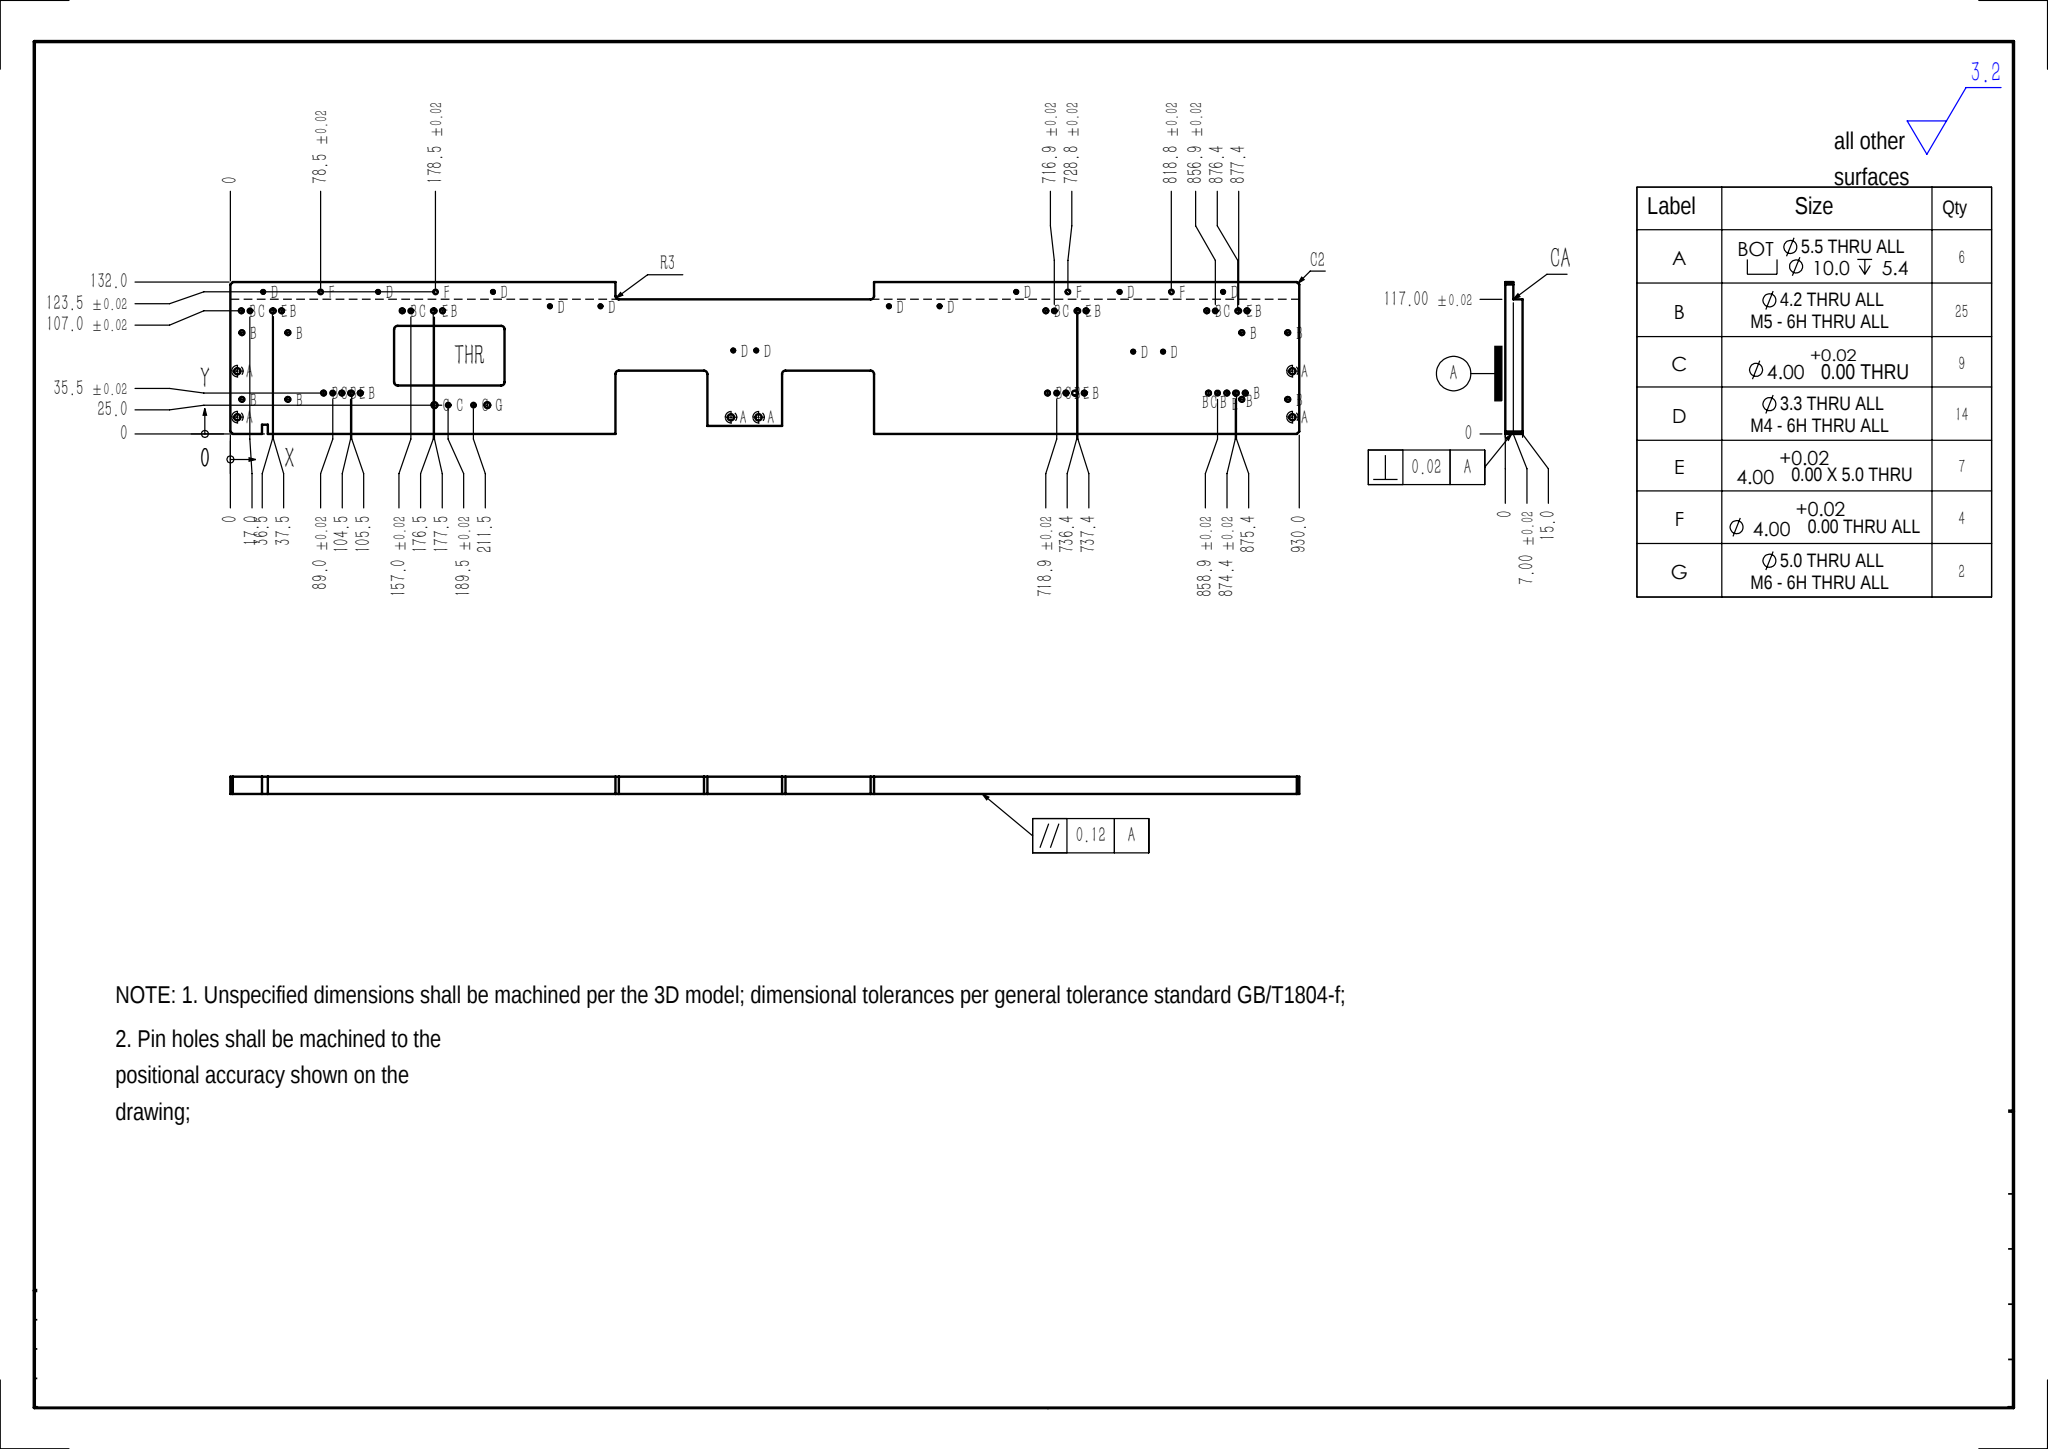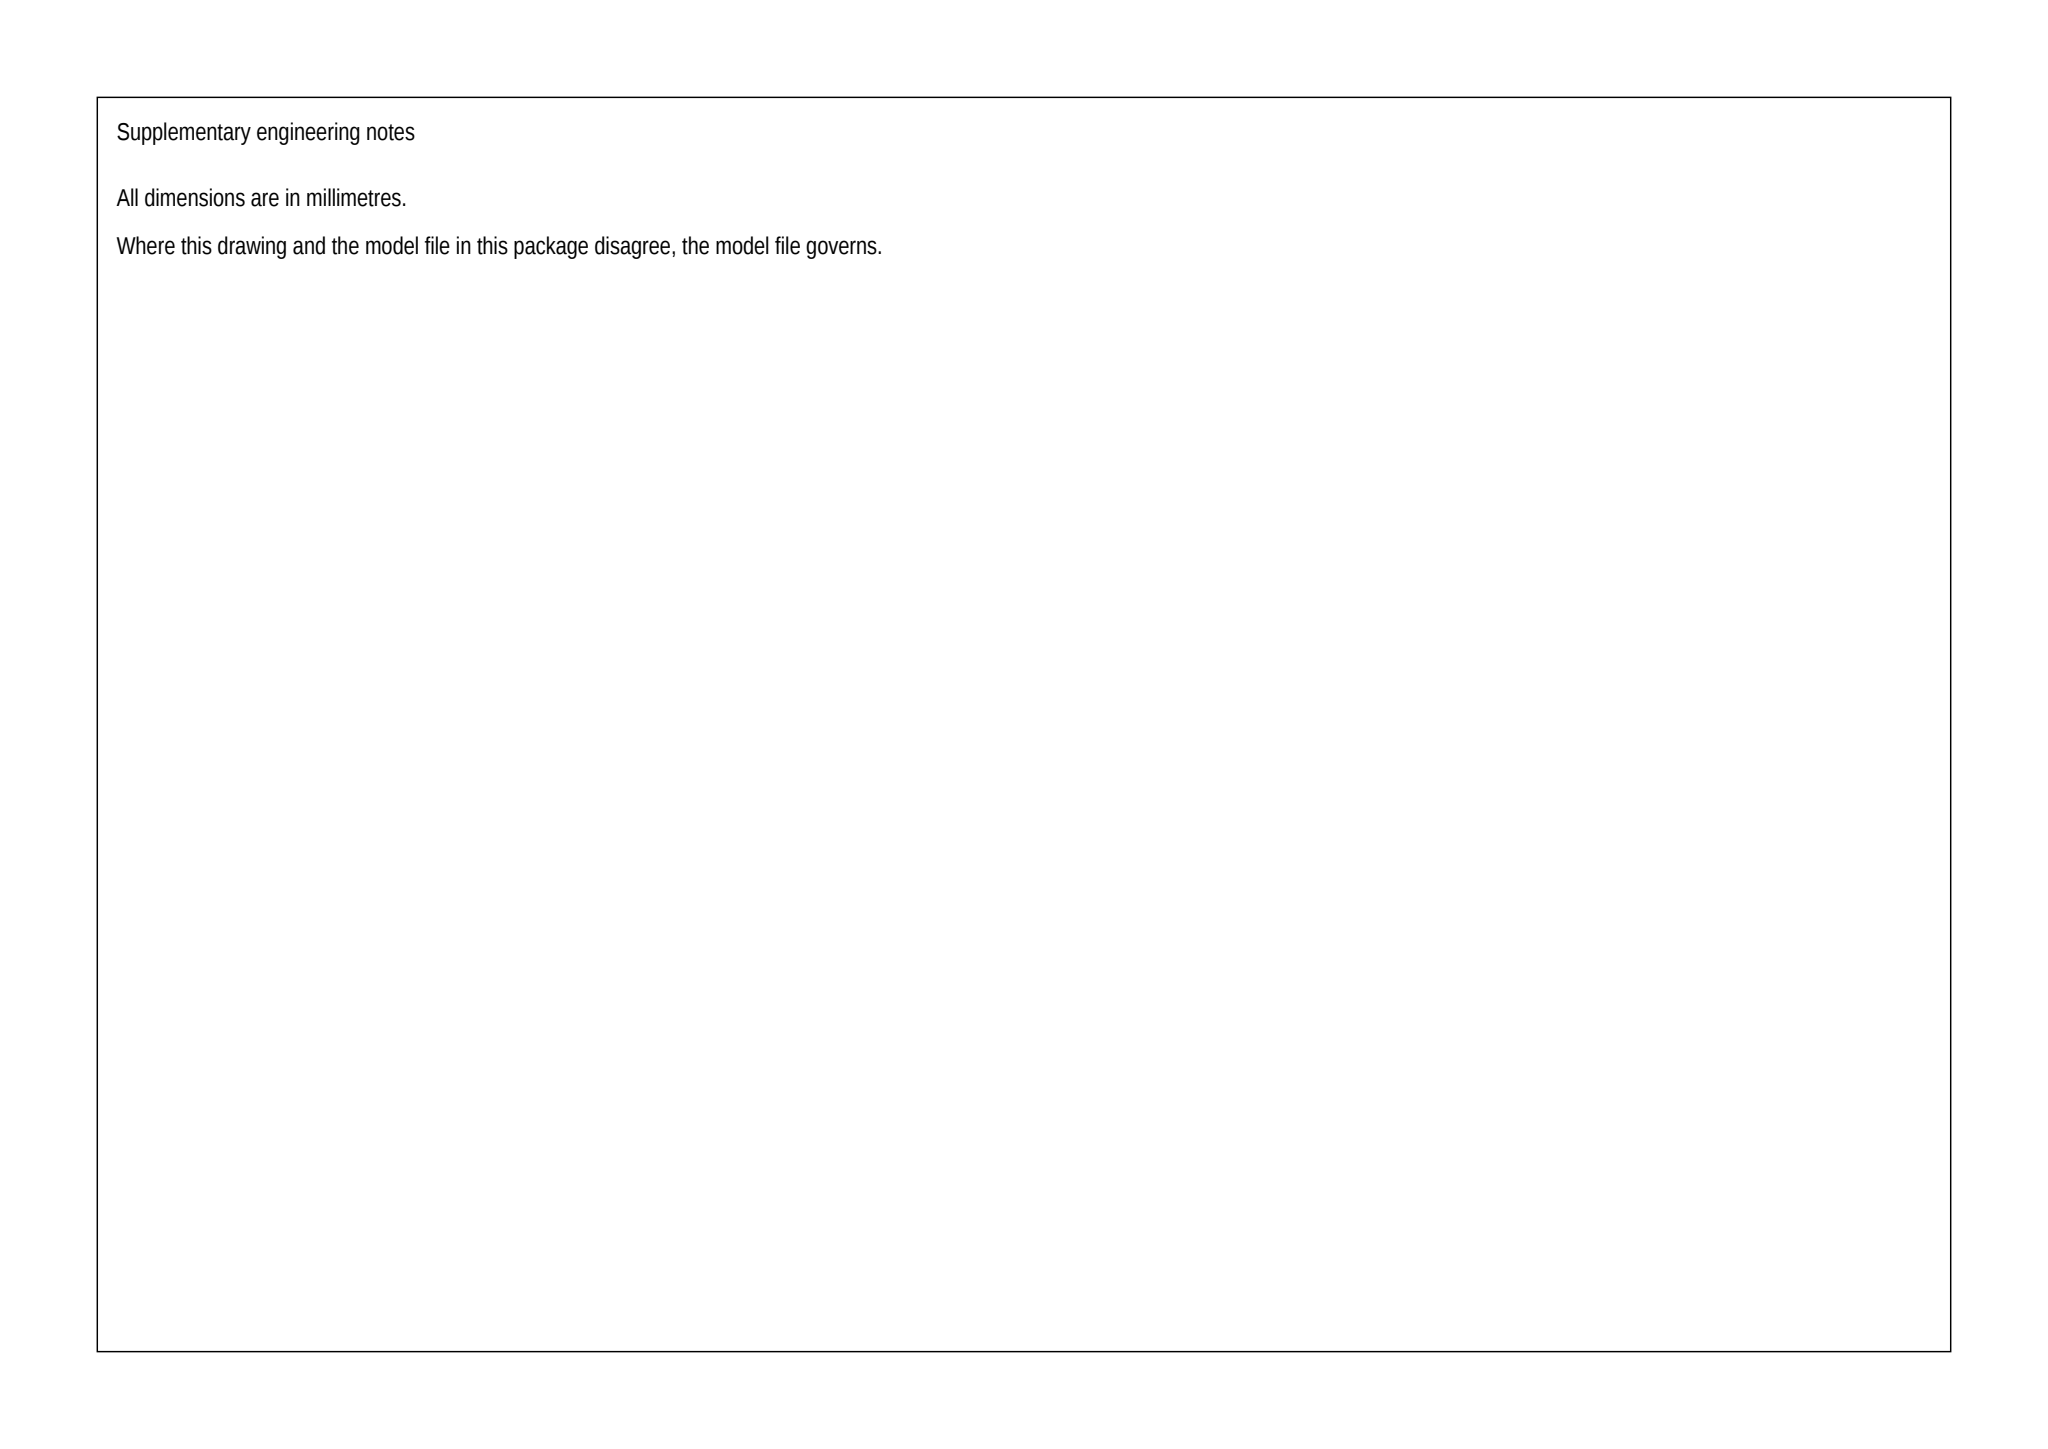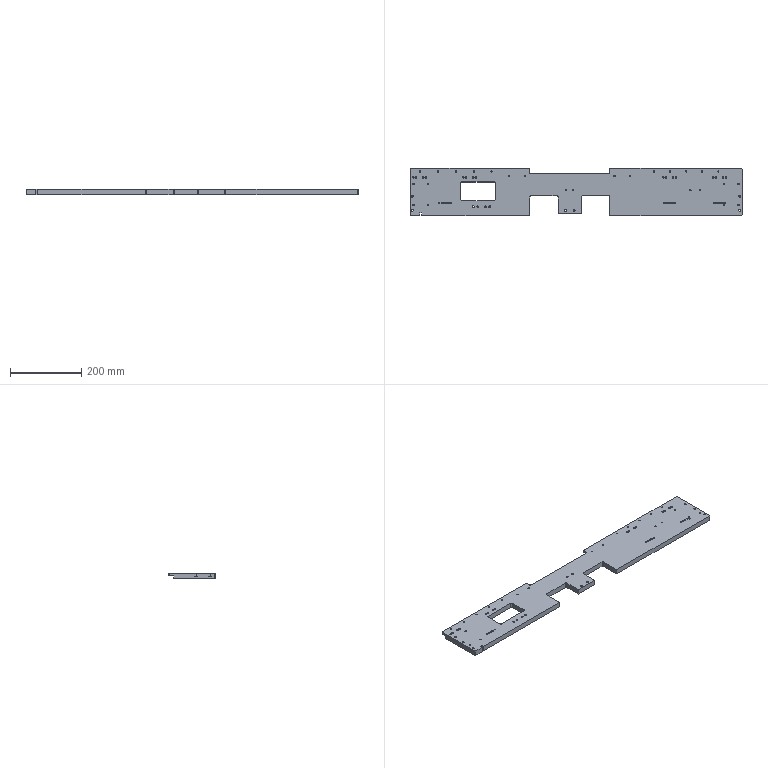Part | SolidWorks | mm | 1 solid | 215 faces | box 930 x 132 x 15 mm | volume 1477170 mm3 | cylinder 163 | plane 52 | commonest cylinder face diameters 4.2 x50 4 x47 3.3 x28 10 x12 5.5 x12 6 x10 5 x4
build123d program:
from build123d import *

# Parameters (mm, degrees)
SKETCH1_W                                       = 930
SKETCH1_H                                       = 132
BOSS_EXTRUDE1_DEPTH                             = 15
SKETCH3_W                                       = 930
SKETCH3_H                                       = 8
CUT_EXTRUDE2_DEPTH                              = 15
SKETCH19_W                                      = 80
SKETCH19_H                                      = 55
SKETCH19_W_2                                    = 225
SKETCH19_H_2                                    = 15
CUT_EXTRUDE3_DEPTH                              = 470.9
SKETCH20_W                                      = 65
SKETCH20_H                                      = 7
CUT_EXTRUDE4_DEPTH                              = 470.9
SKETCH22_W                                      = 96
SKETCH22_H                                      = 52
CUT_EXTRUDE5_DEPTH                              = 470.9
FILLET1_R                                       = 3
M4_TAPPED_HOLE1_D                               = 3.3
M5_TAPPED_HOLE1_D                               = 4.2
M6_TAPPED_HOLE1_D                               = 5
SKETCH29_R                                      = 2
CUT_EXTRUDE6_DEPTH                              = 470.9
CHAMFER1_SIZE                                   = 2
M5_TAPPED_HOLE2_D                               = 4.2
M5_HEX_SOCKET_HEAD_CAP_SCREW_CBORE1_D           = 5.5
M5_HEX_SOCKET_HEAD_CAP_SCREW_CBORE1_CBORE_D     = 10
M5_HEX_SOCKET_HEAD_CAP_SCREW_CBORE1_CBORE_DEPTH = 5.4
M5_HEX_SOCKET_HEAD_CAP_SCREW_CBORE2_D           = 5.5
M5_HEX_SOCKET_HEAD_CAP_SCREW_CBORE2_CBORE_D     = 10
M5_HEX_SOCKET_HEAD_CAP_SCREW_CBORE2_CBORE_DEPTH = 5.4
M5_TAPPED_HOLE3_D                               = 4.2
SKETCH41_W                                      = 5
SKETCH41_H                                      = 8
CUT_EXTRUDE7_DEPTH                              = 470.9
M4_TAPPED_HOLE3_D                               = 3.3
SIZE_MM_DOWEL_HOLE1_D                           = 4


with BuildPart() as part:
    # Sketch1 → Boss-Extrude1 (new body)
    with BuildSketch(Plane.XY):
        Rectangle(SKETCH1_W, SKETCH1_H)
    extrude(amount=BOSS_EXTRUDE1_DEPTH)

    # Sketch3 → Cut-Extrude2 (cut)
    with BuildSketch(Plane(origin=(0, 66, 0), x_dir=(1, 0, 0), z_dir=(0, 1, 0))):
        with Locations((0, -4)):
            Rectangle(SKETCH3_W, SKETCH3_H)
    extrude(amount=-CUT_EXTRUDE2_DEPTH, mode=Mode.SUBTRACT)

    # Sketch19 → Cut-Extrude3 (cut, through all)
    with BuildSketch(Plane.XY.offset(15)):
        with Locations((-90, -38.5)):
            Rectangle(SKETCH19_W, SKETCH19_H)
        with Locations((55, -38.5)):
            Rectangle(SKETCH19_W, SKETCH19_H)
        with Locations((-17.5, 58.5)):
            Rectangle(SKETCH19_W_2, SKETCH19_H_2)
    extrude(amount=-CUT_EXTRUDE3_DEPTH, mode=Mode.SUBTRACT)

    # Sketch20 → Cut-Extrude4 (cut, through all)
    with BuildSketch(Plane.XY.offset(15)):
        with Locations((-17.5, -62.5)):
            Rectangle(SKETCH20_W, SKETCH20_H)
    extrude(amount=-CUT_EXTRUDE4_DEPTH, mode=Mode.SUBTRACT)

    # Sketch22 → Cut-Extrude5 (cut, through all)
    with BuildSketch(Plane.XY.offset(15)):
        with Locations((-274.5, 2)):
            Rectangle(SKETCH22_W, SKETCH22_H)
    extrude(amount=-CUT_EXTRUDE5_DEPTH, mode=Mode.SUBTRACT)

    # Fillet1
    fillet1_edges = [part.edges().sort_by_distance(p)[0] for p in [
        (-226.5, 28, 7.5),
        (-226.5, -24, 7.5),
        (95, 51, 11.5),
        (-130, 51, 11.5),
        (15, -11, 7.5),
        (95, -11, 7.5),
        (-130, -11, 7.5),
        (-50, -11, 7.5),
        (-322.5, -24, 7.5),
        (-322.5, 28, 7.5),
    ]]
    fillet(fillet1_edges, radius=FILLET1_R)

    # M4 Tapped Hole1 (through all)
    with Locations(Plane.XY.offset(15)):
        with Locations((-187, 45), (-143, 45), (-27.5, 6.5), (-7.5, 6.5), (108, 45), (152, 45), (320.5, 5.5), (346.5, 5.5)):
            Hole(M4_TAPPED_HOLE1_D / 2)

    # M5 Tapped Hole1 (through all)
    with Locations(Plane.XY.offset(15)):
        with Locations((-384, -30.5), (-368, -30.5), (-352, -30.5), (246, -30.5), (262, -30.5), (278, -30.5), (386, -30.5), (402, -30.5), (418, -30.5)):
            Hole(M5_TAPPED_HOLE1_D / 2)

    # M6 Tapped Hole1 (through all)
    with Locations(Plane.XY.offset(15)):
        with Locations((-287.5, -41), (-241.5, -41)):
            Hole(M6_TAPPED_HOLE1_D / 2)

    # Sketch29 → Cut-Extrude6 (cut, through all)
    with BuildSketch(Plane.XY.offset(15)):
        with Locations((-376, -30.5)):
            Circle(SKETCH29_R)
        with Locations((-275.5, -41)):
            Circle(SKETCH29_R)
        with Locations((-253.5, -41)):
            Circle(SKETCH29_R)
        with Locations((253.922, -30.5)):
            Circle(SKETCH29_R)
        with Locations((393.922, -30.5)):
            Circle(SKETCH29_R)
        with Locations((-448, 41)):
            Circle(SKETCH29_R)
        with Locations((-308, 41)):
            Circle(SKETCH29_R)
        with Locations((251.922, 41)):
            Circle(SKETCH29_R)
        with Locations((391.922, 41)):
            Circle(SKETCH29_R)
        with BuildLine():
            Line((-360.5, -28.5), (-359.5, -28.5))
            ThreePointArc((-359.5, -28.5), (-357.5, -30.5), (-359.5, -32.5))
            Line((-359.5, -32.5), (-360.5, -32.5))
            ThreePointArc((-360.5, -32.5), (-362.5, -30.5), (-360.5, -28.5))
        make_face()
        with BuildLine():
            Line((269.422, -28.5), (270.422, -28.5))
            ThreePointArc((270.422, -28.5), (272.422, -30.5), (270.422, -32.5))
            Line((270.422, -32.5), (269.422, -32.5))
            ThreePointArc((269.422, -32.5), (267.422, -30.5), (269.422, -28.5))
        make_face()
        with BuildLine():
            Line((409.422, -28.5), (410.422, -28.5))
            ThreePointArc((410.422, -28.5), (412.422, -30.5), (410.422, -32.5))
            Line((410.422, -32.5), (409.422, -32.5))
            ThreePointArc((409.422, -32.5), (407.422, -30.5), (409.422, -28.5))
        make_face()
        with BuildLine():
            Line((-428.5, 43), (-427.5, 43))
            ThreePointArc((-427.5, 43), (-425.5, 41), (-427.5, 39))
            Line((-427.5, 39), (-428.5, 39))
            ThreePointArc((-428.5, 39), (-430.5, 41), (-428.5, 43))
        make_face()
        with BuildLine():
            Line((-288.5, 43), (-287.5, 43))
            ThreePointArc((-287.5, 43), (-285.5, 41), (-287.5, 39))
            Line((-287.5, 39), (-288.5, 39))
            ThreePointArc((-288.5, 39), (-290.5, 41), (-288.5, 43))
        make_face()
        with BuildLine():
            Line((271.422, 43), (272.422, 43))
            ThreePointArc((272.422, 43), (274.422, 41), (272.422, 39))
            Line((272.422, 39), (271.422, 39))
            ThreePointArc((271.422, 39), (269.422, 41), (271.422, 43))
        make_face()
        with BuildLine():
            Line((411.422, 43), (412.422, 43))
            ThreePointArc((412.422, 43), (414.422, 41), (412.422, 39))
            Line((412.422, 39), (411.422, 39))
            ThreePointArc((411.422, 39), (409.422, 41), (411.422, 43))
        make_face()
    extrude(amount=-CUT_EXTRUDE6_DEPTH, mode=Mode.SUBTRACT)

    # Chamfer1
    chamfer1_edges = [part.edges().sort_by_distance(p)[0] for p in [
        (-465, 66, 11.5),
        (465, 66, 11.5),
        (465, -66, 7.5),
        (-465, -66, 7.5),
    ]]
    chamfer(chamfer1_edges, length=CHAMFER1_SIZE)

    # M5 Tapped Hole2 (through all)
    with Locations(Plane.XY.offset(15)):
        with Locations((-455.5, 41), (-420.5, 41), (-315.5, 41), (-280.5, 41), (244.5, 41), (279.5, 41), (384.5, 41), (419.5, 41)):
            Hole(M5_TAPPED_HOLE2_D / 2)

    # M5 Hex Socket Head Cap Screw CBORE1 (through all)
    with Locations(Plane(origin=(0, 0, 0), x_dir=(-1, 0, 0), z_dir=(0, 0, -1))):
        with Locations((5.5, -51.6), (29.5, -51.6)):
            CounterBoreHole(M5_HEX_SOCKET_HEAD_CAP_SCREW_CBORE1_D / 2, M5_HEX_SOCKET_HEAD_CAP_SCREW_CBORE1_CBORE_D / 2, M5_HEX_SOCKET_HEAD_CAP_SCREW_CBORE1_CBORE_DEPTH)

    # M5 Hex Socket Head Cap Screw CBORE2 (through all)
    with Locations(Plane(origin=(0, 0, 0), x_dir=(-1, 0, 0), z_dir=(0, 0, -1))):
        with Locations((459, -11.5), (459, -51.5)):
            m5_hex_socket_head_cap_screw_cbore2 = CounterBoreHole(M5_HEX_SOCKET_HEAD_CAP_SCREW_CBORE2_D / 2, M5_HEX_SOCKET_HEAD_CAP_SCREW_CBORE2_CBORE_D / 2, M5_HEX_SOCKET_HEAD_CAP_SCREW_CBORE2_CBORE_DEPTH)

    # M5 Tapped Hole3 (through all)
    with Locations(Plane(origin=(0, 0, 0), x_dir=(-1, 0, 0), z_dir=(0, 0, -1))):
        with Locations((415, 22), (455, 22), (415, -36), (455, -36)):
            m5_tapped_hole3 = Hole(M5_TAPPED_HOLE3_D / 2)

    # Mirror1: M5 Hex Socket Head Cap Screw CBORE2, M5 Tapped Hole3 across plane
    add(m5_hex_socket_head_cap_screw_cbore2.mirror(Plane(origin=(0, 0, 0), x_dir=(0, 0, 1), z_dir=(1, 0, 0))), mode=Mode.SUBTRACT)
    add(m5_tapped_hole3.mirror(Plane(origin=(0, 0, 0), x_dir=(0, 0, 1), z_dir=(1, 0, 0))), mode=Mode.SUBTRACT)

    # Sketch41 → Cut-Extrude7 (cut, through all)
    with BuildSketch(Plane(origin=(0, 0, 0), x_dir=(-1, 0, 0), z_dir=(0, 0, -1))):
        with Locations((435, -62)):
            Rectangle(SKETCH41_W, SKETCH41_H)
    extrude(amount=-CUT_EXTRUDE7_DEPTH, mode=Mode.SUBTRACT)

    # M4 Tapped Hole3 (through all)
    with Locations(Plane(origin=(0, 0, 8), x_dir=(-1, 0, 0), z_dir=(0, 0, -1))):
        with Locations((-398.75, 57.5), (-308.75, 57.5), (-218.75, 57.5), (236.5, 57.5), (336.5, 57.5), (436.5, 57.5)):
            Hole(M4_TAPPED_HOLE3_D / 2)

    # Size mm Dowel Hole1 (through all)
    with Locations(Plane(origin=(0, 0, 8), x_dir=(-1, 0, 0), z_dir=(0, 0, -1))):
        with Locations((-353.75, 57.5), (-263.75, 57.5), (286.5, 57.5), (386.5, 57.5)):
            Hole(SIZE_MM_DOWEL_HOLE1_D / 2)


solid = part.part